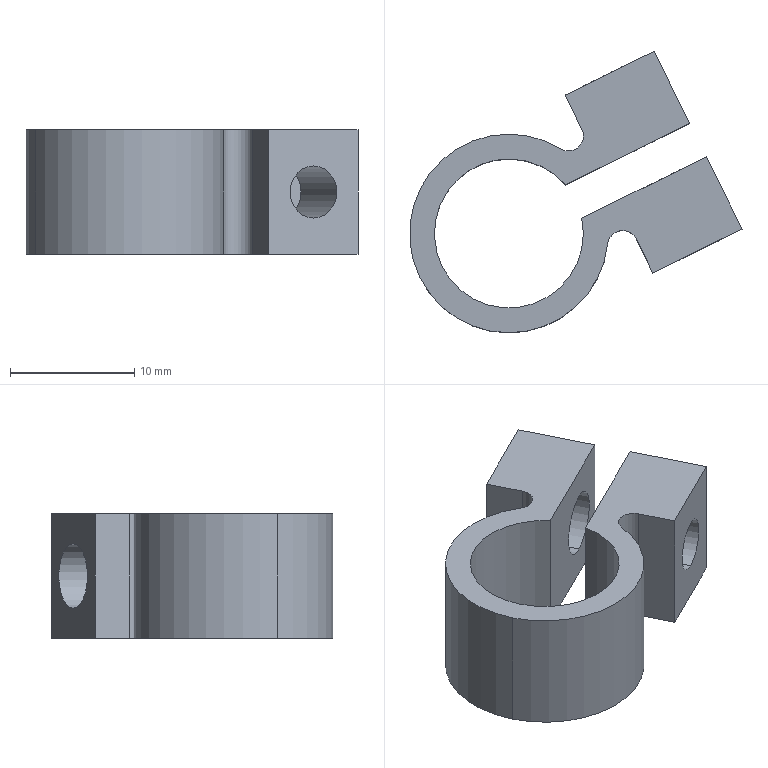Component | SolidWorks | TAR-02-038ShaftClampBlock-2 | 1 solid | 20 faces | box 26.79 x 22.7 x 10 mm | volume 1704 mm3 | cylinder 10 | plane 10 | commonest cylinder face diameters 4.2 x2 5.2 x2 16 x2 12 x2 2.43 x2
build123d program:
from build123d import *

# Parameters (mm, degrees)
BOSS_EXTRUDE1_DEPTH = 10
SKETCH2_R           = 2.6
CUT_EXTRUDE1_DEPTH  = 8
M5_TAPPED_HOLE1_D   = 4.2


with BuildPart() as part:
    # Sketch1 → Boss-Extrude1 (new body)
    with BuildSketch(Plane.XY):
        with BuildLine():
            Line((9, 8), (17, 8))
            Line((17, 8), (17, 1.5))
            Line((17, 1.5), (5.809, 1.5))
            ThreePointArc((5.809, 1.5), (-6, 0), (5.809, -1.5))
            Line((5.809, -1.5), (17, -1.5))
            Line((17, -1.5), (17, -8))
            Line((17, -8), (9, -8))
            Line((9, -8), (9, -4.93))
            ThreePointArc((9, -4.93), (8.124, -3.763), (6.759, -4.28))
            ThreePointArc((6.759, -4.28), (-8, 0), (6.759, 4.28))
            ThreePointArc((6.759, 4.28), (8.124, 3.763), (9, 4.93))
            Line((9, 4.93), (9, 8))
        make_face()
    extrude(amount=BOSS_EXTRUDE1_DEPTH)

    # Sketch2 → Cut-Extrude1 (cut)
    with BuildSketch(Plane(origin=(0, 8, 0), x_dir=(1, 0, 0), z_dir=(0, 1, 0))):
        with Locations(Location((13, -5, 0), (0, 0, 270))):
            Circle(SKETCH2_R)
    extrude(amount=-CUT_EXTRUDE1_DEPTH, mode=Mode.SUBTRACT)

    # M5 Tapped Hole1 (through all)
    with Locations(Plane(origin=(13, 8, 5), x_dir=(0, 0, 1), z_dir=(0, 1, 0))):
        with Locations((0, 0)):
            Hole(M5_TAPPED_HOLE1_D / 2)


solid = part.part

# Placed as in the assembly
solid = solid.moved(Location((-115.391, 9.288, -57.94), (0, 0, 26.267)))
STEP:
#1=COLOUR_RGB('',0.7922,0.8196,0.9333);
#2=FILL_AREA_STYLE_COLOUR('',#1);
#3=FILL_AREA_STYLE('',(#2));
#4=SURFACE_STYLE_FILL_AREA(#3);
#5=SURFACE_SIDE_STYLE('',(#4));
#6=SURFACE_STYLE_USAGE(.BOTH.,#5);
#7=PRESENTATION_STYLE_ASSIGNMENT((#6));
#8=CARTESIAN_POINT('',(-3.945,0.3097,-2.167));
#9=VERTEX_POINT('',#8);
#10=CARTESIAN_POINT('',(-3.945,0.3097,-2.002));
#11=VERTEX_POINT('',#10);
#12=CARTESIAN_POINT('',(-3.945,0.3097,-2.084));
#13=DIRECTION('',(-0.4425,0.8967,0.));
#14=DIRECTION('',(0.,0.,1.));
#15=AXIS2_PLACEMENT_3D('',#12,#13,#14);
#16=CIRCLE('',#15,0.08268);
#17=EDGE_CURVE('',#9,#11,#16,.T.);
#18=ORIENTED_EDGE('',*,*,#17,.F.);
#19=CARTESIAN_POINT('',(-4.058,0.5392,-2.167));
#20=VERTEX_POINT('',#19);
#21=CARTESIAN_POINT('',(-4.223,0.8746,-2.167));
#22=DIRECTION('',(-0.4425,0.8967,0.));
#23=VECTOR('',#22,39.37);
#24=LINE('',#21,#23);
#25=EDGE_CURVE('',#9,#20,#24,.T.);
#26=ORIENTED_EDGE('',*,*,#25,.T.);
#27=CARTESIAN_POINT('',(-4.058,0.5392,-2.002));
#28=VERTEX_POINT('',#27);
#29=CARTESIAN_POINT('',(-4.058,0.5392,-2.084));
#30=DIRECTION('',(0.4425,-0.8967,0.));
#31=DIRECTION('',(0.8967,0.4425,0.));
#32=AXIS2_PLACEMENT_3D('',#29,#30,#31);
#33=CIRCLE('',#32,0.08268);
#34=EDGE_CURVE('',#28,#20,#33,.T.);
#35=ORIENTED_EDGE('',*,*,#34,.F.);
#36=CARTESIAN_POINT('',(-4.223,0.8746,-2.002));
#37=DIRECTION('',(-0.4425,0.8967,0.));
#38=VECTOR('',#37,39.37);
#39=LINE('',#36,#38);
#40=EDGE_CURVE('',#11,#28,#39,.T.);
#41=ORIENTED_EDGE('',*,*,#40,.F.);
#42=EDGE_LOOP('',(#18,#26,#35,#41));
#43=FACE_OUTER_BOUND('',#42,.T.);
#44=CARTESIAN_POINT('',(-4.223,0.8746,-2.084));
#45=DIRECTION('',(-0.4425,0.8967,0.));
#46=DIRECTION('',(0.,0.,1.));
#47=AXIS2_PLACEMENT_3D('',#44,#45,#46);
#48=CYLINDRICAL_SURFACE('',#47,0.08268);
#49=ADVANCED_FACE('',(#43),#48,.F.);
#50=CARTESIAN_POINT('',(-4.11,0.6451,-2.187));
#51=VERTEX_POINT('',#50);
#52=CARTESIAN_POINT('',(-4.11,0.6451,-1.982));
#53=VERTEX_POINT('',#52);
#54=CARTESIAN_POINT('',(-4.11,0.6451,-2.084));
#55=DIRECTION('',(-0.4425,0.8967,0.));
#56=DIRECTION('',(-0.8967,-0.4425,0.));
#57=AXIS2_PLACEMENT_3D('',#54,#55,#56);
#58=CIRCLE('',#57,0.1024);
#59=EDGE_CURVE('',#51,#53,#58,.T.);
#60=ORIENTED_EDGE('',*,*,#59,.F.);
#61=CARTESIAN_POINT('',(-4.223,0.8746,-2.187));
#62=VERTEX_POINT('',#61);
#63=CARTESIAN_POINT('',(-4.084,0.5922,-2.187));
#64=DIRECTION('',(-0.4425,0.8967,0.));
#65=VECTOR('',#64,39.37);
#66=LINE('',#63,#65);
#67=EDGE_CURVE('',#51,#62,#66,.T.);
#68=ORIENTED_EDGE('',*,*,#67,.T.);
#69=CARTESIAN_POINT('',(-4.223,0.8746,-1.982));
#70=VERTEX_POINT('',#69);
#71=CARTESIAN_POINT('',(-4.223,0.8746,-2.084));
#72=DIRECTION('',(-0.4425,0.8967,0.));
#73=DIRECTION('',(0.,0.,1.));
#74=AXIS2_PLACEMENT_3D('',#71,#72,#73);
#75=CIRCLE('',#74,0.1024);
#76=EDGE_CURVE('',#62,#70,#75,.T.);
#77=ORIENTED_EDGE('',*,*,#76,.T.);
#78=CARTESIAN_POINT('',(-4.084,0.5922,-1.982));
#79=DIRECTION('',(-0.4425,0.8967,0.));
#80=VECTOR('',#79,39.37);
#81=LINE('',#78,#80);
#82=EDGE_CURVE('',#53,#70,#81,.T.);
#83=ORIENTED_EDGE('',*,*,#82,.F.);
#84=EDGE_LOOP('',(#60,#68,#77,#83));
#85=FACE_OUTER_BOUND('',#84,.T.);
#86=CARTESIAN_POINT('',(-4.084,0.5922,-2.084));
#87=DIRECTION('',(-0.4425,0.8967,0.));
#88=DIRECTION('',(0.,0.,1.));
#89=AXIS2_PLACEMENT_3D('',#86,#87,#88);
#90=CYLINDRICAL_SURFACE('',#89,0.1024);
#91=ADVANCED_FACE('',(#85),#90,.F.);
#92=CARTESIAN_POINT('',(-4.825,0.2263,-1.887));
#93=VERTEX_POINT('',#92);
#94=CARTESIAN_POINT('',(-4.23,0.3323,-1.887));
#95=VERTEX_POINT('',#94);
#96=CARTESIAN_POINT('',(-4.543,0.3657,-1.887));
#97=DIRECTION('',(0.,0.,1.));
#98=DIRECTION('',(0.8967,0.4425,0.));
#99=AXIS2_PLACEMENT_3D('',#96,#97,#98);
#100=CIRCLE('',#99,0.315);
#101=EDGE_CURVE('',#93,#95,#100,.T.);
#102=ORIENTED_EDGE('',*,*,#101,.F.);
#103=CARTESIAN_POINT('',(-4.825,0.2263,-2.281));
#104=VERTEX_POINT('',#103);
#105=CARTESIAN_POINT('',(-4.825,0.2263,-1.887));
#106=DIRECTION('',(0.,0.,-1.));
#107=VECTOR('',#106,39.37);
#108=LINE('',#105,#107);
#109=EDGE_CURVE('',#93,#104,#108,.T.);
#110=ORIENTED_EDGE('',*,*,#109,.T.);
#111=CARTESIAN_POINT('',(-4.23,0.3323,-2.281));
#112=VERTEX_POINT('',#111);
#113=CARTESIAN_POINT('',(-4.543,0.3657,-2.281));
#114=DIRECTION('',(0.,0.,1.));
#115=DIRECTION('',(0.8967,0.4425,0.));
#116=AXIS2_PLACEMENT_3D('',#113,#114,#115);
#117=CIRCLE('',#116,0.315);
#118=EDGE_CURVE('',#104,#112,#117,.T.);
#119=ORIENTED_EDGE('',*,*,#118,.T.);
#120=CARTESIAN_POINT('',(-4.23,0.3323,-1.887));
#121=DIRECTION('',(0.,0.,-1.));
#122=VECTOR('',#121,39.37);
#123=LINE('',#120,#122);
#124=EDGE_CURVE('',#95,#112,#123,.T.);
#125=ORIENTED_EDGE('',*,*,#124,.F.);
#126=EDGE_LOOP('',(#102,#110,#119,#125));
#127=FACE_OUTER_BOUND('',#126,.T.);
#128=CARTESIAN_POINT('',(-4.543,0.3657,-1.887));
#129=DIRECTION('',(0.,0.,-1.));
#130=DIRECTION('',(-0.8967,-0.4425,0.));
#131=AXIS2_PLACEMENT_3D('',#128,#129,#130);
#132=CYLINDRICAL_SURFACE('',#131,0.315);
#133=ADVANCED_FACE('',(#127),#132,.T.);
#134=CARTESIAN_POINT('',(-4.755,0.2611,-1.887));
#135=VERTEX_POINT('',#134);
#136=CARTESIAN_POINT('',(-4.364,0.5198,-1.887));
#137=VERTEX_POINT('',#136);
#138=CARTESIAN_POINT('',(-4.543,0.3657,-1.887));
#139=DIRECTION('',(0.,0.,-1.));
#140=DIRECTION('',(0.8967,0.4425,0.));
#141=AXIS2_PLACEMENT_3D('',#138,#139,#140);
#142=CIRCLE('',#141,0.2362);
#143=EDGE_CURVE('',#135,#137,#142,.T.);
#144=ORIENTED_EDGE('',*,*,#143,.F.);
#145=CARTESIAN_POINT('',(-4.755,0.2611,-2.281));
#146=VERTEX_POINT('',#145);
#147=CARTESIAN_POINT('',(-4.755,0.2611,-1.887));
#148=DIRECTION('',(0.,0.,-1.));
#149=VECTOR('',#148,39.37);
#150=LINE('',#147,#149);
#151=EDGE_CURVE('',#135,#146,#150,.T.);
#152=ORIENTED_EDGE('',*,*,#151,.T.);
#153=CARTESIAN_POINT('',(-4.364,0.5198,-2.281));
#154=VERTEX_POINT('',#153);
#155=CARTESIAN_POINT('',(-4.543,0.3657,-2.281));
#156=DIRECTION('',(0.,0.,-1.));
#157=DIRECTION('',(0.8967,0.4425,0.));
#158=AXIS2_PLACEMENT_3D('',#155,#156,#157);
#159=CIRCLE('',#158,0.2362);
#160=EDGE_CURVE('',#146,#154,#159,.T.);
#161=ORIENTED_EDGE('',*,*,#160,.T.);
#162=CARTESIAN_POINT('',(-4.364,0.5198,-1.887));
#163=DIRECTION('',(0.,0.,-1.));
#164=VECTOR('',#163,39.37);
#165=LINE('',#162,#164);
#166=EDGE_CURVE('',#137,#154,#165,.T.);
#167=ORIENTED_EDGE('',*,*,#166,.F.);
#168=EDGE_LOOP('',(#144,#152,#161,#167));
#169=FACE_OUTER_BOUND('',#168,.T.);
#170=CARTESIAN_POINT('',(-4.543,0.3657,-1.887));
#171=DIRECTION('',(0.,0.,-1.));
#172=DIRECTION('',(-0.8967,-0.4425,0.));
#173=AXIS2_PLACEMENT_3D('',#170,#171,#172);
#174=CYLINDRICAL_SURFACE('',#173,0.2362);
#175=ADVANCED_FACE('',(#169),#174,.F.);
#176=CARTESIAN_POINT('',(-4.139,0.3484,-2.281));
#177=VERTEX_POINT('',#176);
#178=CARTESIAN_POINT('',(-4.182,0.3272,-2.281));
#179=DIRECTION('',(0.,0.,-1.));
#180=DIRECTION('',(-0.8967,-0.4425,0.));
#181=AXIS2_PLACEMENT_3D('',#178,#179,#180);
#182=CIRCLE('',#181,0.04783);
#183=EDGE_CURVE('',#112,#177,#182,.T.);
#184=ORIENTED_EDGE('',*,*,#183,.T.);
#185=CARTESIAN_POINT('',(-4.139,0.3484,-1.887));
#186=VERTEX_POINT('',#185);
#187=CARTESIAN_POINT('',(-4.139,0.3484,-1.887));
#188=DIRECTION('',(0.,0.,-1.));
#189=VECTOR('',#188,39.37);
#190=LINE('',#187,#189);
#191=EDGE_CURVE('',#186,#177,#190,.T.);
#192=ORIENTED_EDGE('',*,*,#191,.F.);
#193=CARTESIAN_POINT('',(-4.182,0.3272,-1.887));
#194=DIRECTION('',(0.,0.,-1.));
#195=DIRECTION('',(-0.8967,-0.4425,0.));
#196=AXIS2_PLACEMENT_3D('',#193,#194,#195);
#197=CIRCLE('',#196,0.04783);
#198=EDGE_CURVE('',#95,#186,#197,.T.);
#199=ORIENTED_EDGE('',*,*,#198,.F.);
#200=ORIENTED_EDGE('',*,*,#124,.T.);
#201=EDGE_LOOP('',(#184,#192,#199,#200));
#202=FACE_OUTER_BOUND('',#201,.T.);
#203=CARTESIAN_POINT('',(-4.182,0.3272,-1.887));
#204=DIRECTION('',(0.,0.,-1.));
#205=DIRECTION('',(-0.8967,-0.4425,0.));
#206=AXIS2_PLACEMENT_3D('',#203,#204,#205);
#207=CYLINDRICAL_SURFACE('',#206,0.04783);
#208=ADVANCED_FACE('',(#202),#207,.F.);
#209=CARTESIAN_POINT('',(-4.086,0.24,-2.281));
#210=VERTEX_POINT('',#209);
#211=CARTESIAN_POINT('',(-4.086,0.24,-2.281));
#212=DIRECTION('',(0.4425,-0.8967,0.));
#213=VECTOR('',#212,39.37);
#214=LINE('',#211,#213);
#215=EDGE_CURVE('',#177,#210,#214,.T.);
#216=ORIENTED_EDGE('',*,*,#215,.T.);
#217=CARTESIAN_POINT('',(-4.086,0.24,-1.887));
#218=VERTEX_POINT('',#217);
#219=CARTESIAN_POINT('',(-4.086,0.24,-1.887));
#220=DIRECTION('',(0.,0.,-1.));
#221=VECTOR('',#220,39.37);
#222=LINE('',#219,#221);
#223=EDGE_CURVE('',#218,#210,#222,.T.);
#224=ORIENTED_EDGE('',*,*,#223,.F.);
#225=CARTESIAN_POINT('',(-4.086,0.24,-1.887));
#226=DIRECTION('',(0.4425,-0.8967,0.));
#227=VECTOR('',#226,39.37);
#228=LINE('',#225,#227);
#229=EDGE_CURVE('',#186,#218,#228,.T.);
#230=ORIENTED_EDGE('',*,*,#229,.F.);
#231=ORIENTED_EDGE('',*,*,#191,.T.);
#232=EDGE_LOOP('',(#216,#224,#230,#231));
#233=FACE_OUTER_BOUND('',#232,.T.);
#234=CARTESIAN_POINT('',(-4.086,0.24,-1.887));
#235=DIRECTION('',(0.8967,0.4425,0.));
#236=DIRECTION('',(0.,0.,-1.));
#237=AXIS2_PLACEMENT_3D('',#234,#235,#236);
#238=PLANE('',#237);
#239=ADVANCED_FACE('',(#233),#238,.F.);
#240=CARTESIAN_POINT('',(-3.945,0.3097,-2.084));
#241=DIRECTION('',(-0.4425,0.8967,0.));
#242=DIRECTION('',(0.,0.,1.));
#243=AXIS2_PLACEMENT_3D('',#240,#241,#242);
#244=CIRCLE('',#243,0.08268);
#245=EDGE_CURVE('',#11,#9,#244,.T.);
#246=ORIENTED_EDGE('',*,*,#245,.T.);
#247=ORIENTED_EDGE('',*,*,#17,.T.);
#248=EDGE_LOOP('',(#246,#247));
#249=FACE_BOUND('',#248,.T.);
#250=CARTESIAN_POINT('',(-3.803,0.3794,-2.281));
#251=VERTEX_POINT('',#250);
#252=CARTESIAN_POINT('',(-3.803,0.3794,-2.281));
#253=DIRECTION('',(0.8967,0.4425,0.));
#254=VECTOR('',#253,39.37);
#255=LINE('',#252,#254);
#256=EDGE_CURVE('',#210,#251,#255,.T.);
#257=ORIENTED_EDGE('',*,*,#256,.T.);
#258=CARTESIAN_POINT('',(-3.803,0.3794,-1.887));
#259=VERTEX_POINT('',#258);
#260=CARTESIAN_POINT('',(-3.803,0.3794,-1.887));
#261=DIRECTION('',(0.,0.,-1.));
#262=VECTOR('',#261,39.37);
#263=LINE('',#260,#262);
#264=EDGE_CURVE('',#259,#251,#263,.T.);
#265=ORIENTED_EDGE('',*,*,#264,.F.);
#266=CARTESIAN_POINT('',(-3.803,0.3794,-1.887));
#267=DIRECTION('',(0.8967,0.4425,0.));
#268=VECTOR('',#267,39.37);
#269=LINE('',#266,#268);
#270=EDGE_CURVE('',#218,#259,#269,.T.);
#271=ORIENTED_EDGE('',*,*,#270,.F.);
#272=ORIENTED_EDGE('',*,*,#223,.T.);
#273=EDGE_LOOP('',(#257,#265,#271,#272));
#274=FACE_OUTER_BOUND('',#273,.T.);
#275=CARTESIAN_POINT('',(-3.803,0.3794,-1.887));
#276=DIRECTION('',(-0.4425,0.8967,0.));
#277=DIRECTION('',(-0.8967,-0.4425,0.));
#278=AXIS2_PLACEMENT_3D('',#275,#276,#277);
#279=PLANE('',#278);
#280=ADVANCED_FACE('',(#249,#274),#279,.F.);
#281=CARTESIAN_POINT('',(-3.917,0.6089,-2.281));
#282=VERTEX_POINT('',#281);
#283=CARTESIAN_POINT('',(-3.917,0.6089,-2.281));
#284=DIRECTION('',(-0.4425,0.8967,0.));
#285=VECTOR('',#284,39.37);
#286=LINE('',#283,#285);
#287=EDGE_CURVE('',#251,#282,#286,.T.);
#288=ORIENTED_EDGE('',*,*,#287,.T.);
#289=CARTESIAN_POINT('',(-3.917,0.6089,-1.887));
#290=VERTEX_POINT('',#289);
#291=CARTESIAN_POINT('',(-3.917,0.6089,-1.887));
#292=DIRECTION('',(0.,0.,-1.));
#293=VECTOR('',#292,39.37);
#294=LINE('',#291,#293);
#295=EDGE_CURVE('',#290,#282,#294,.T.);
#296=ORIENTED_EDGE('',*,*,#295,.F.);
#297=CARTESIAN_POINT('',(-3.917,0.6089,-1.887));
#298=DIRECTION('',(-0.4425,0.8967,0.));
#299=VECTOR('',#298,39.37);
#300=LINE('',#297,#299);
#301=EDGE_CURVE('',#259,#290,#300,.T.);
#302=ORIENTED_EDGE('',*,*,#301,.F.);
#303=ORIENTED_EDGE('',*,*,#264,.T.);
#304=EDGE_LOOP('',(#288,#296,#302,#303));
#305=FACE_OUTER_BOUND('',#304,.T.);
#306=CARTESIAN_POINT('',(-3.917,0.6089,-1.887));
#307=DIRECTION('',(-0.8967,-0.4425,0.));
#308=DIRECTION('',(0.,0.,1.));
#309=AXIS2_PLACEMENT_3D('',#306,#307,#308);
#310=PLANE('',#309);
#311=ADVANCED_FACE('',(#305),#310,.F.);
#312=ORIENTED_EDGE('',*,*,#34,.T.);
#313=CARTESIAN_POINT('',(-4.058,0.5392,-2.084));
#314=DIRECTION('',(0.4425,-0.8967,0.));
#315=DIRECTION('',(0.8967,0.4425,0.));
#316=AXIS2_PLACEMENT_3D('',#313,#314,#315);
#317=CIRCLE('',#316,0.08268);
#318=EDGE_CURVE('',#20,#28,#317,.T.);
#319=ORIENTED_EDGE('',*,*,#318,.T.);
#320=EDGE_LOOP('',(#312,#319));
#321=FACE_BOUND('',#320,.T.);
#322=CARTESIAN_POINT('',(-4.312,0.4139,-2.281));
#323=VERTEX_POINT('',#322);
#324=CARTESIAN_POINT('',(-4.312,0.4139,-2.281));
#325=DIRECTION('',(-0.8967,-0.4425,0.));
#326=VECTOR('',#325,39.37);
#327=LINE('',#324,#326);
#328=EDGE_CURVE('',#282,#323,#327,.T.);
#329=ORIENTED_EDGE('',*,*,#328,.T.);
#330=CARTESIAN_POINT('',(-4.312,0.4139,-1.887));
#331=VERTEX_POINT('',#330);
#332=CARTESIAN_POINT('',(-4.312,0.4139,-1.887));
#333=DIRECTION('',(0.,0.,-1.));
#334=VECTOR('',#333,39.37);
#335=LINE('',#332,#334);
#336=EDGE_CURVE('',#331,#323,#335,.T.);
#337=ORIENTED_EDGE('',*,*,#336,.F.);
#338=CARTESIAN_POINT('',(-4.312,0.4139,-1.887));
#339=DIRECTION('',(-0.8967,-0.4425,0.));
#340=VECTOR('',#339,39.37);
#341=LINE('',#338,#340);
#342=EDGE_CURVE('',#290,#331,#341,.T.);
#343=ORIENTED_EDGE('',*,*,#342,.F.);
#344=ORIENTED_EDGE('',*,*,#295,.T.);
#345=EDGE_LOOP('',(#329,#337,#343,#344));
#346=FACE_OUTER_BOUND('',#345,.T.);
#347=CARTESIAN_POINT('',(-4.312,0.4139,-1.887));
#348=DIRECTION('',(0.4425,-0.8967,0.));
#349=DIRECTION('',(0.8967,0.4425,0.));
#350=AXIS2_PLACEMENT_3D('',#347,#348,#349);
#351=PLANE('',#350);
#352=ADVANCED_FACE('',(#321,#346),#351,.F.);
#353=ORIENTED_EDGE('',*,*,#151,.F.);
#354=CARTESIAN_POINT('',(-4.543,0.3657,-1.887));
#355=DIRECTION('',(0.,0.,-1.));
#356=DIRECTION('',(0.8967,0.4425,0.));
#357=AXIS2_PLACEMENT_3D('',#354,#355,#356);
#358=CIRCLE('',#357,0.2362);
#359=EDGE_CURVE('',#331,#135,#358,.T.);
#360=ORIENTED_EDGE('',*,*,#359,.F.);
#361=ORIENTED_EDGE('',*,*,#336,.T.);
#362=CARTESIAN_POINT('',(-4.543,0.3657,-2.281));
#363=DIRECTION('',(0.,0.,-1.));
#364=DIRECTION('',(0.8967,0.4425,0.));
#365=AXIS2_PLACEMENT_3D('',#362,#363,#364);
#366=CIRCLE('',#365,0.2362);
#367=EDGE_CURVE('',#323,#146,#366,.T.);
#368=ORIENTED_EDGE('',*,*,#367,.T.);
#369=EDGE_LOOP('',(#353,#360,#361,#368));
#370=FACE_OUTER_BOUND('',#369,.T.);
#371=CARTESIAN_POINT('',(-4.543,0.3657,-1.887));
#372=DIRECTION('',(0.,0.,-1.));
#373=DIRECTION('',(-0.8967,-0.4425,0.));
#374=AXIS2_PLACEMENT_3D('',#371,#372,#373);
#375=CYLINDRICAL_SURFACE('',#374,0.2362);
#376=ADVANCED_FACE('',(#370),#375,.F.);
#377=CARTESIAN_POINT('',(-4.11,0.6451,-2.084));
#378=DIRECTION('',(-0.4425,0.8967,0.));
#379=DIRECTION('',(-0.8967,-0.4425,0.));
#380=AXIS2_PLACEMENT_3D('',#377,#378,#379);
#381=CIRCLE('',#380,0.1024);
#382=EDGE_CURVE('',#53,#51,#381,.T.);
#383=ORIENTED_EDGE('',*,*,#382,.T.);
#384=ORIENTED_EDGE('',*,*,#59,.T.);
#385=EDGE_LOOP('',(#383,#384));
#386=FACE_BOUND('',#385,.T.);
#387=CARTESIAN_POINT('',(-3.969,0.7148,-2.281));
#388=VERTEX_POINT('',#387);
#389=CARTESIAN_POINT('',(-4.364,0.5198,-2.281));
#390=DIRECTION('',(0.8967,0.4425,0.));
#391=VECTOR('',#390,39.37);
#392=LINE('',#389,#391);
#393=EDGE_CURVE('',#154,#388,#392,.T.);
#394=ORIENTED_EDGE('',*,*,#393,.T.);
#395=CARTESIAN_POINT('',(-3.969,0.7148,-1.887));
#396=VERTEX_POINT('',#395);
#397=CARTESIAN_POINT('',(-3.969,0.7148,-1.887));
#398=DIRECTION('',(0.,0.,-1.));
#399=VECTOR('',#398,39.37);
#400=LINE('',#397,#399);
#401=EDGE_CURVE('',#396,#388,#400,.T.);
#402=ORIENTED_EDGE('',*,*,#401,.F.);
#403=CARTESIAN_POINT('',(-4.364,0.5198,-1.887));
#404=DIRECTION('',(0.8967,0.4425,0.));
#405=VECTOR('',#404,39.37);
#406=LINE('',#403,#405);
#407=EDGE_CURVE('',#137,#396,#406,.T.);
#408=ORIENTED_EDGE('',*,*,#407,.F.);
#409=ORIENTED_EDGE('',*,*,#166,.T.);
#410=EDGE_LOOP('',(#394,#402,#408,#409));
#411=FACE_OUTER_BOUND('',#410,.T.);
#412=CARTESIAN_POINT('',(-4.364,0.5198,-1.887));
#413=DIRECTION('',(-0.4425,0.8967,0.));
#414=DIRECTION('',(-0.8967,-0.4425,0.));
#415=AXIS2_PLACEMENT_3D('',#412,#413,#414);
#416=PLANE('',#415);
#417=ADVANCED_FACE('',(#386,#411),#416,.F.);
#418=CARTESIAN_POINT('',(-4.082,0.9443,-2.281));
#419=VERTEX_POINT('',#418);
#420=CARTESIAN_POINT('',(-4.082,0.9443,-2.281));
#421=DIRECTION('',(-0.4425,0.8967,0.));
#422=VECTOR('',#421,39.37);
#423=LINE('',#420,#422);
#424=EDGE_CURVE('',#388,#419,#423,.T.);
#425=ORIENTED_EDGE('',*,*,#424,.T.);
#426=CARTESIAN_POINT('',(-4.082,0.9443,-1.887));
#427=VERTEX_POINT('',#426);
#428=CARTESIAN_POINT('',(-4.082,0.9443,-1.887));
#429=DIRECTION('',(0.,0.,-1.));
#430=VECTOR('',#429,39.37);
#431=LINE('',#428,#430);
#432=EDGE_CURVE('',#427,#419,#431,.T.);
#433=ORIENTED_EDGE('',*,*,#432,.F.);
#434=CARTESIAN_POINT('',(-4.082,0.9443,-1.887));
#435=DIRECTION('',(-0.4425,0.8967,0.));
#436=VECTOR('',#435,39.37);
#437=LINE('',#434,#436);
#438=EDGE_CURVE('',#396,#427,#437,.T.);
#439=ORIENTED_EDGE('',*,*,#438,.F.);
#440=ORIENTED_EDGE('',*,*,#401,.T.);
#441=EDGE_LOOP('',(#425,#433,#439,#440));
#442=FACE_OUTER_BOUND('',#441,.T.);
#443=CARTESIAN_POINT('',(-4.082,0.9443,-1.887));
#444=DIRECTION('',(-0.8967,-0.4425,0.));
#445=DIRECTION('',(0.,0.,1.));
#446=AXIS2_PLACEMENT_3D('',#443,#444,#445);
#447=PLANE('',#446);
#448=ADVANCED_FACE('',(#442),#447,.F.);
#449=CARTESIAN_POINT('',(-4.223,0.8746,-2.084));
#450=DIRECTION('',(-0.4425,0.8967,0.));
#451=DIRECTION('',(0.,0.,1.));
#452=AXIS2_PLACEMENT_3D('',#449,#450,#451);
#453=CIRCLE('',#452,0.1024);
#454=EDGE_CURVE('',#70,#62,#453,.T.);
#455=ORIENTED_EDGE('',*,*,#454,.F.);
#456=ORIENTED_EDGE('',*,*,#76,.F.);
#457=EDGE_LOOP('',(#455,#456));
#458=FACE_BOUND('',#457,.T.);
#459=CARTESIAN_POINT('',(-4.365,0.8049,-2.281));
#460=VERTEX_POINT('',#459);
#461=CARTESIAN_POINT('',(-4.365,0.8049,-2.281));
#462=DIRECTION('',(-0.8967,-0.4425,0.));
#463=VECTOR('',#462,39.37);
#464=LINE('',#461,#463);
#465=EDGE_CURVE('',#419,#460,#464,.T.);
#466=ORIENTED_EDGE('',*,*,#465,.T.);
#467=CARTESIAN_POINT('',(-4.365,0.8049,-1.887));
#468=VERTEX_POINT('',#467);
#469=CARTESIAN_POINT('',(-4.365,0.8049,-1.887));
#470=DIRECTION('',(0.,0.,-1.));
#471=VECTOR('',#470,39.37);
#472=LINE('',#469,#471);
#473=EDGE_CURVE('',#468,#460,#472,.T.);
#474=ORIENTED_EDGE('',*,*,#473,.F.);
#475=CARTESIAN_POINT('',(-4.365,0.8049,-1.887));
#476=DIRECTION('',(-0.8967,-0.4425,0.));
#477=VECTOR('',#476,39.37);
#478=LINE('',#475,#477);
#479=EDGE_CURVE('',#427,#468,#478,.T.);
#480=ORIENTED_EDGE('',*,*,#479,.F.);
#481=ORIENTED_EDGE('',*,*,#432,.T.);
#482=EDGE_LOOP('',(#466,#474,#480,#481));
#483=FACE_OUTER_BOUND('',#482,.T.);
#484=CARTESIAN_POINT('',(-4.365,0.8049,-1.887));
#485=DIRECTION('',(0.4425,-0.8967,0.));
#486=DIRECTION('',(0.,0.,-1.));
#487=AXIS2_PLACEMENT_3D('',#484,#485,#486);
#488=PLANE('',#487);
#489=ADVANCED_FACE('',(#458,#483),#488,.F.);
#490=CARTESIAN_POINT('',(-4.311,0.6965,-2.281));
#491=VERTEX_POINT('',#490);
#492=CARTESIAN_POINT('',(-4.311,0.6965,-2.281));
#493=DIRECTION('',(0.4425,-0.8967,0.));
#494=VECTOR('',#493,39.37);
#495=LINE('',#492,#494);
#496=EDGE_CURVE('',#460,#491,#495,.T.);
#497=ORIENTED_EDGE('',*,*,#496,.T.);
#498=CARTESIAN_POINT('',(-4.311,0.6965,-1.887));
#499=VERTEX_POINT('',#498);
#500=CARTESIAN_POINT('',(-4.311,0.6965,-1.887));
#501=DIRECTION('',(0.,0.,-1.));
#502=VECTOR('',#501,39.37);
#503=LINE('',#500,#502);
#504=EDGE_CURVE('',#499,#491,#503,.T.);
#505=ORIENTED_EDGE('',*,*,#504,.F.);
#506=CARTESIAN_POINT('',(-4.311,0.6965,-1.887));
#507=DIRECTION('',(0.4425,-0.8967,0.));
#508=VECTOR('',#507,39.37);
#509=LINE('',#506,#508);
#510=EDGE_CURVE('',#468,#499,#509,.T.);
#511=ORIENTED_EDGE('',*,*,#510,.F.);
#512=ORIENTED_EDGE('',*,*,#473,.T.);
#513=EDGE_LOOP('',(#497,#505,#511,#512));
#514=FACE_OUTER_BOUND('',#513,.T.);
#515=CARTESIAN_POINT('',(-4.311,0.6965,-1.887));
#516=DIRECTION('',(0.8967,0.4425,0.));
#517=DIRECTION('',(0.,0.,-1.));
#518=AXIS2_PLACEMENT_3D('',#515,#516,#517);
#519=PLANE('',#518);
#520=ADVANCED_FACE('',(#514),#519,.F.);
#521=CARTESIAN_POINT('',(-4.379,0.6345,-2.281));
#522=VERTEX_POINT('',#521);
#523=CARTESIAN_POINT('',(-4.354,0.6754,-2.281));
#524=DIRECTION('',(0.,0.,-1.));
#525=DIRECTION('',(0.8967,0.4425,0.));
#526=AXIS2_PLACEMENT_3D('',#523,#524,#525);
#527=CIRCLE('',#526,0.04783);
#528=EDGE_CURVE('',#491,#522,#527,.T.);
#529=ORIENTED_EDGE('',*,*,#528,.T.);
#530=CARTESIAN_POINT('',(-4.379,0.6345,-1.887));
#531=VERTEX_POINT('',#530);
#532=CARTESIAN_POINT('',(-4.379,0.6345,-1.887));
#533=DIRECTION('',(0.,0.,-1.));
#534=VECTOR('',#533,39.37);
#535=LINE('',#532,#534);
#536=EDGE_CURVE('',#531,#522,#535,.T.);
#537=ORIENTED_EDGE('',*,*,#536,.F.);
#538=CARTESIAN_POINT('',(-4.354,0.6754,-1.887));
#539=DIRECTION('',(0.,0.,-1.));
#540=DIRECTION('',(0.8967,0.4425,0.));
#541=AXIS2_PLACEMENT_3D('',#538,#539,#540);
#542=CIRCLE('',#541,0.04783);
#543=EDGE_CURVE('',#499,#531,#542,.T.);
#544=ORIENTED_EDGE('',*,*,#543,.F.);
#545=ORIENTED_EDGE('',*,*,#504,.T.);
#546=EDGE_LOOP('',(#529,#537,#544,#545));
#547=FACE_OUTER_BOUND('',#546,.T.);
#548=CARTESIAN_POINT('',(-4.354,0.6754,-1.887));
#549=DIRECTION('',(0.,0.,-1.));
#550=DIRECTION('',(-0.8967,-0.4425,0.));
#551=AXIS2_PLACEMENT_3D('',#548,#549,#550);
#552=CYLINDRICAL_SURFACE('',#551,0.04783);
#553=ADVANCED_FACE('',(#547),#552,.F.);
#554=ORIENTED_EDGE('',*,*,#109,.F.);
#555=CARTESIAN_POINT('',(-4.543,0.3657,-1.887));
#556=DIRECTION('',(0.,0.,1.));
#557=DIRECTION('',(0.8967,0.4425,0.));
#558=AXIS2_PLACEMENT_3D('',#555,#556,#557);
#559=CIRCLE('',#558,0.315);
#560=EDGE_CURVE('',#531,#93,#559,.T.);
#561=ORIENTED_EDGE('',*,*,#560,.F.);
#562=ORIENTED_EDGE('',*,*,#536,.T.);
#563=CARTESIAN_POINT('',(-4.543,0.3657,-2.281));
#564=DIRECTION('',(0.,0.,1.));
#565=DIRECTION('',(0.8967,0.4425,0.));
#566=AXIS2_PLACEMENT_3D('',#563,#564,#565);
#567=CIRCLE('',#566,0.315);
#568=EDGE_CURVE('',#522,#104,#567,.T.);
#569=ORIENTED_EDGE('',*,*,#568,.T.);
#570=EDGE_LOOP('',(#554,#561,#562,#569));
#571=FACE_OUTER_BOUND('',#570,.T.);
#572=CARTESIAN_POINT('',(-4.543,0.3657,-1.887));
#573=DIRECTION('',(0.,0.,-1.));
#574=DIRECTION('',(-0.8967,-0.4425,0.));
#575=AXIS2_PLACEMENT_3D('',#572,#573,#574);
#576=CYLINDRICAL_SURFACE('',#575,0.315);
#577=ADVANCED_FACE('',(#571),#576,.T.);
#578=ORIENTED_EDGE('',*,*,#198,.T.);
#579=ORIENTED_EDGE('',*,*,#229,.T.);
#580=ORIENTED_EDGE('',*,*,#270,.T.);
#581=ORIENTED_EDGE('',*,*,#301,.T.);
#582=ORIENTED_EDGE('',*,*,#342,.T.);
#583=ORIENTED_EDGE('',*,*,#359,.T.);
#584=ORIENTED_EDGE('',*,*,#143,.T.);
#585=ORIENTED_EDGE('',*,*,#407,.T.);
#586=ORIENTED_EDGE('',*,*,#438,.T.);
#587=ORIENTED_EDGE('',*,*,#479,.T.);
#588=ORIENTED_EDGE('',*,*,#510,.T.);
#589=ORIENTED_EDGE('',*,*,#543,.T.);
#590=ORIENTED_EDGE('',*,*,#560,.T.);
#591=ORIENTED_EDGE('',*,*,#101,.T.);
#592=EDGE_LOOP('',(#578,#579,#580,#581,#582,#583,#584,#585,#586,#587,#588,#589,#590,#591));
#593=FACE_OUTER_BOUND('',#592,.T.);
#594=CARTESIAN_POINT('',(-4.182,0.3272,-1.887));
#595=DIRECTION('',(0.,0.,-1.));
#596=DIRECTION('',(-0.8967,-0.4425,0.));
#597=AXIS2_PLACEMENT_3D('',#594,#595,#596);
#598=PLANE('',#597);
#599=ADVANCED_FACE('',(#593),#598,.F.);
#600=ORIENTED_EDGE('',*,*,#183,.F.);
#601=ORIENTED_EDGE('',*,*,#118,.F.);
#602=ORIENTED_EDGE('',*,*,#568,.F.);
#603=ORIENTED_EDGE('',*,*,#528,.F.);
#604=ORIENTED_EDGE('',*,*,#496,.F.);
#605=ORIENTED_EDGE('',*,*,#465,.F.);
#606=ORIENTED_EDGE('',*,*,#424,.F.);
#607=ORIENTED_EDGE('',*,*,#393,.F.);
#608=ORIENTED_EDGE('',*,*,#160,.F.);
#609=ORIENTED_EDGE('',*,*,#367,.F.);
#610=ORIENTED_EDGE('',*,*,#328,.F.);
#611=ORIENTED_EDGE('',*,*,#287,.F.);
#612=ORIENTED_EDGE('',*,*,#256,.F.);
#613=ORIENTED_EDGE('',*,*,#215,.F.);
#614=EDGE_LOOP('',(#600,#601,#602,#603,#604,#605,#606,#607,#608,#609,#610,#611,#612,#613));
#615=FACE_OUTER_BOUND('',#614,.T.);
#616=CARTESIAN_POINT('',(-4.182,0.3272,-2.281));
#617=DIRECTION('',(0.,0.,-1.));
#618=DIRECTION('',(-0.8967,-0.4425,0.));
#619=AXIS2_PLACEMENT_3D('',#616,#617,#618);
#620=PLANE('',#619);
#621=ADVANCED_FACE('',(#615),#620,.T.);
#622=ORIENTED_EDGE('',*,*,#67,.F.);
#623=ORIENTED_EDGE('',*,*,#382,.F.);
#624=ORIENTED_EDGE('',*,*,#82,.T.);
#625=ORIENTED_EDGE('',*,*,#454,.T.);
#626=EDGE_LOOP('',(#622,#623,#624,#625));
#627=FACE_OUTER_BOUND('',#626,.T.);
#628=CARTESIAN_POINT('',(-4.084,0.5922,-2.084));
#629=DIRECTION('',(-0.4425,0.8967,0.));
#630=DIRECTION('',(0.,0.,1.));
#631=AXIS2_PLACEMENT_3D('',#628,#629,#630);
#632=CYLINDRICAL_SURFACE('',#631,0.1024);
#633=ADVANCED_FACE('',(#627),#632,.F.);
#634=ORIENTED_EDGE('',*,*,#25,.F.);
#635=ORIENTED_EDGE('',*,*,#245,.F.);
#636=ORIENTED_EDGE('',*,*,#40,.T.);
#637=ORIENTED_EDGE('',*,*,#318,.F.);
#638=EDGE_LOOP('',(#634,#635,#636,#637));
#639=FACE_OUTER_BOUND('',#638,.T.);
#640=CARTESIAN_POINT('',(-4.223,0.8746,-2.084));
#641=DIRECTION('',(-0.4425,0.8967,0.));
#642=DIRECTION('',(0.,0.,1.));
#643=AXIS2_PLACEMENT_3D('',#640,#641,#642);
#644=CYLINDRICAL_SURFACE('',#643,0.08268);
#645=ADVANCED_FACE('',(#639),#644,.F.);
#646=CLOSED_SHELL('',(#49,#91,#133,#175,#208,#239,#280,#311,#352,#376,#417,#448,#489,#520,#553,#577,#599,#621,#633,#645));
#647=MANIFOLD_SOLID_BREP('',#646);
#648=STYLED_ITEM('',(#7),#647);
#649=PRESENTATION_LAYER_ASSIGNMENT('','',(#648));
#650=(LENGTH_UNIT()NAMED_UNIT(*)SI_UNIT($,.METRE.));
#651=LENGTH_MEASURE_WITH_UNIT(LENGTH_MEASURE(0.0254),#650);
#652=DIMENSIONAL_EXPONENTS(1.,0.,0.,0.,0.,0.,0.);
#653=(CONVERSION_BASED_UNIT('',#651)LENGTH_UNIT()NAMED_UNIT(#652));
#654=UNCERTAINTY_MEASURE_WITH_UNIT(LENGTH_MEASURE(0.00001),#653,'','');
#655=(NAMED_UNIT(*)PLANE_ANGLE_UNIT()SI_UNIT($,.RADIAN.));
#656=(NAMED_UNIT(*)SI_UNIT($,.STERADIAN.)SOLID_ANGLE_UNIT());
#657=(GEOMETRIC_REPRESENTATION_CONTEXT(3)GLOBAL_UNCERTAINTY_ASSIGNED_CONTEXT((#654))GLOBAL_UNIT_ASSIGNED_CONTEXT((#653,#655,#656))REPRESENTATION_CONTEXT('',''));
#658=MECHANICAL_DESIGN_GEOMETRIC_PRESENTATION_REPRESENTATION('',(#648),#657);
#659=CARTESIAN_POINT('',(0.,0.,0.));
#660=DIRECTION('',(0.,0.,1.));
#661=DIRECTION('',(1.,0.,0.));
#662=AXIS2_PLACEMENT_3D('',#659,#660,#661);
#663=(LENGTH_UNIT()NAMED_UNIT(*)SI_UNIT($,.METRE.));
#664=LENGTH_MEASURE_WITH_UNIT(LENGTH_MEASURE(0.0254),#663);
#665=DIMENSIONAL_EXPONENTS(1.,0.,0.,0.,0.,0.,0.);
#666=(CONVERSION_BASED_UNIT('',#664)LENGTH_UNIT()NAMED_UNIT(#665));
#667=UNCERTAINTY_MEASURE_WITH_UNIT(LENGTH_MEASURE(0.00001),#666,'','');
#668=(NAMED_UNIT(*)PLANE_ANGLE_UNIT()SI_UNIT($,.RADIAN.));
#669=(NAMED_UNIT(*)SI_UNIT($,.STERADIAN.)SOLID_ANGLE_UNIT());
#670=(GEOMETRIC_REPRESENTATION_CONTEXT(3)GLOBAL_UNCERTAINTY_ASSIGNED_CONTEXT((#667))GLOBAL_UNIT_ASSIGNED_CONTEXT((#666,#668,#669))REPRESENTATION_CONTEXT('',''));
#671=ADVANCED_BREP_SHAPE_REPRESENTATION('',(#647,#662),#670);